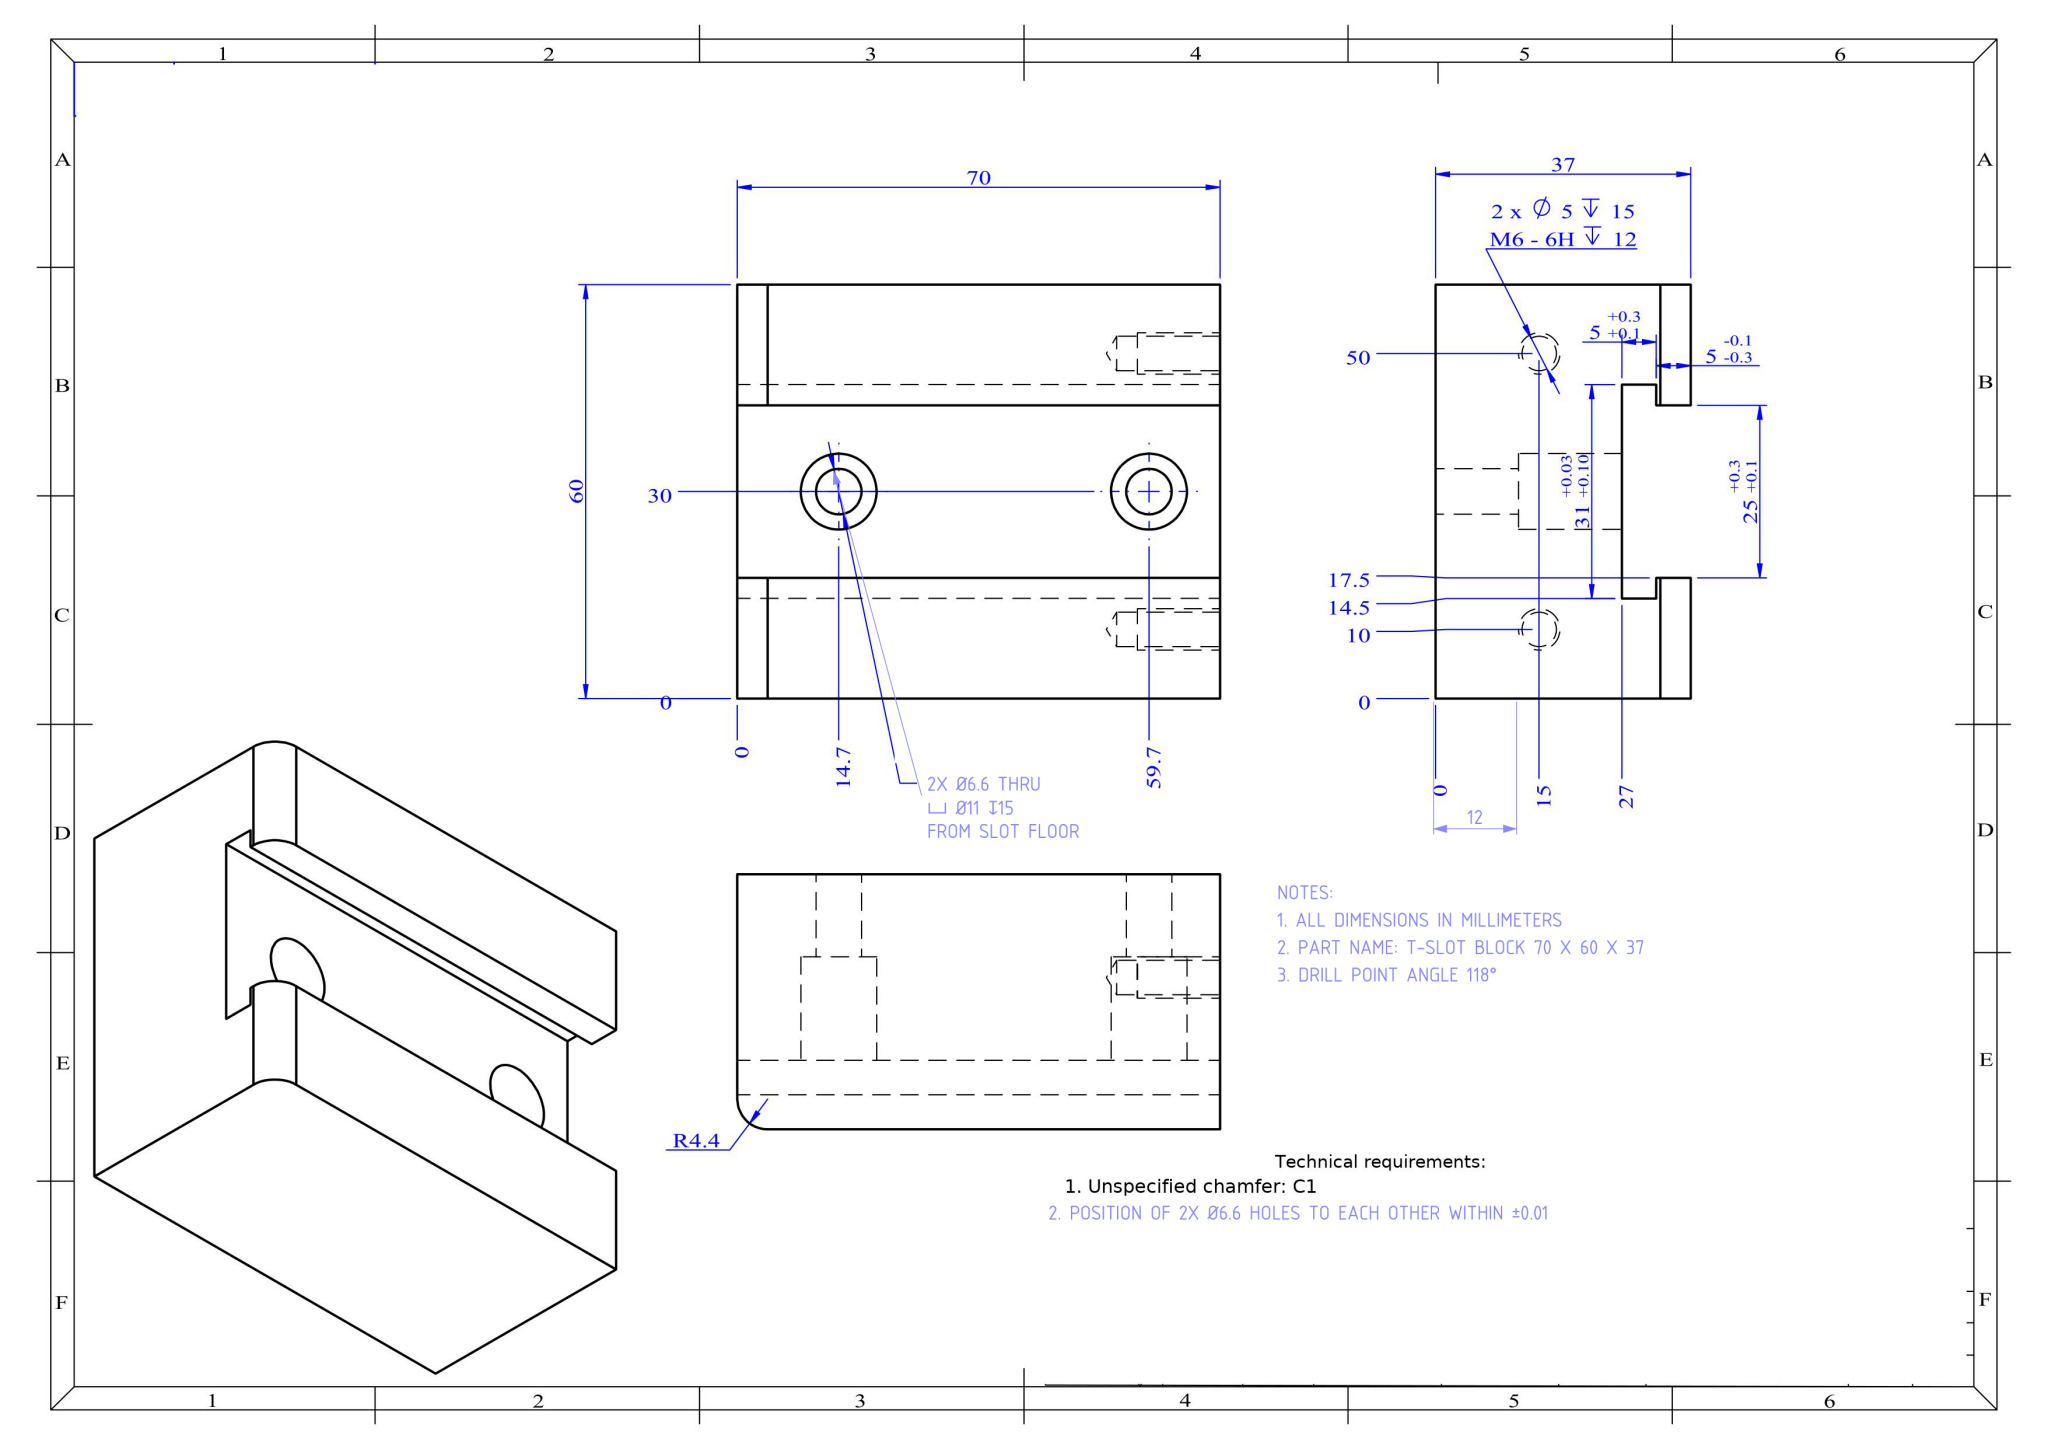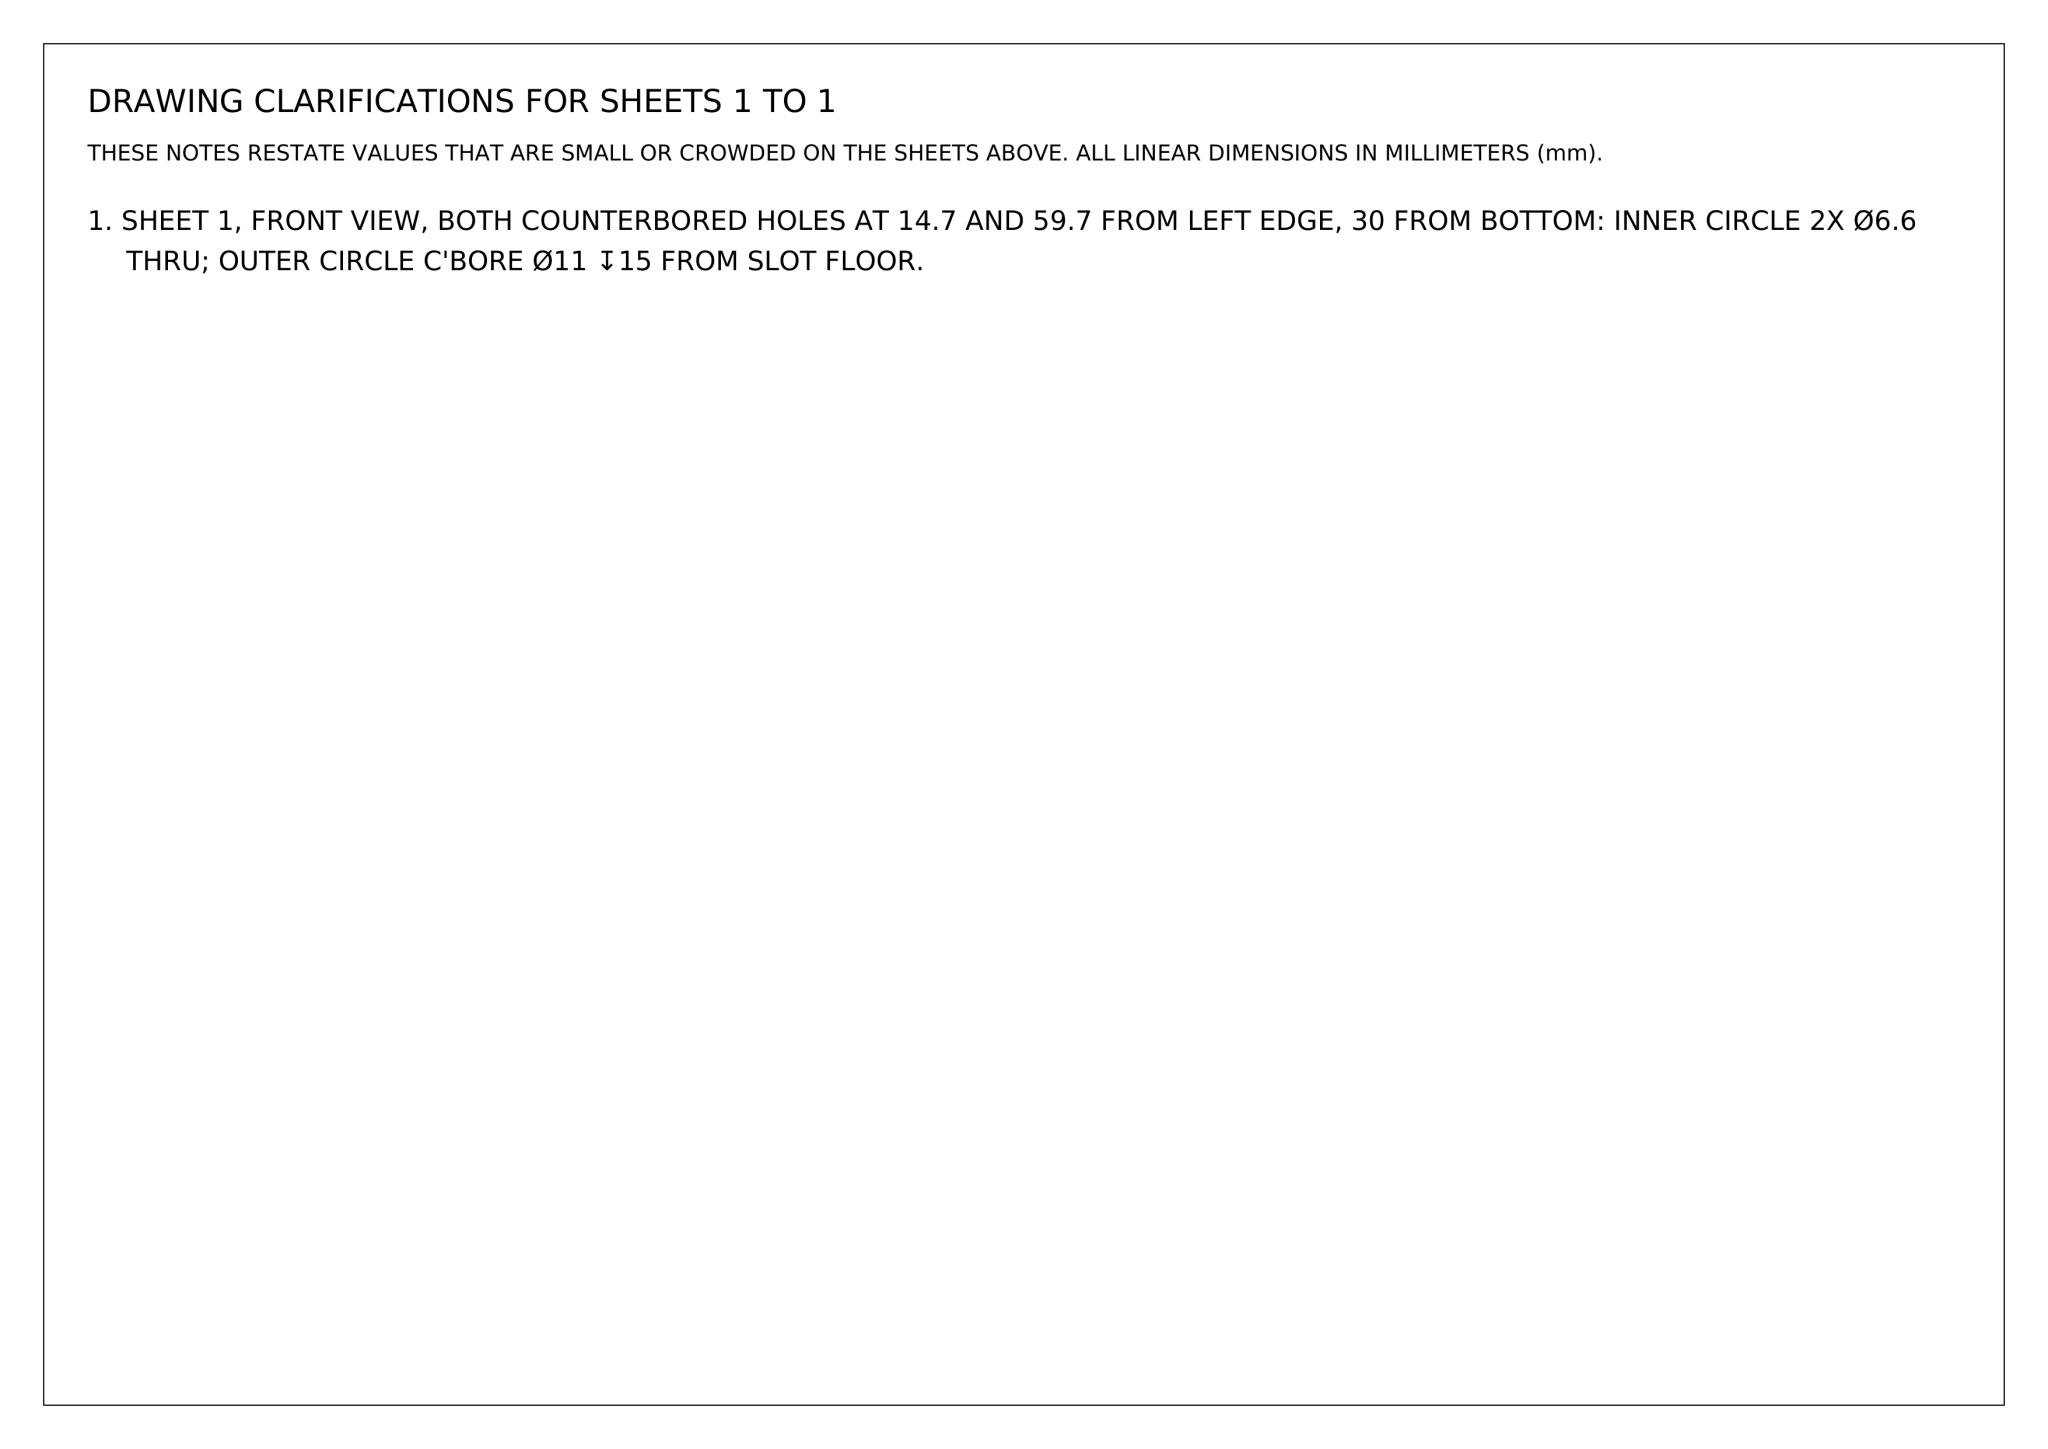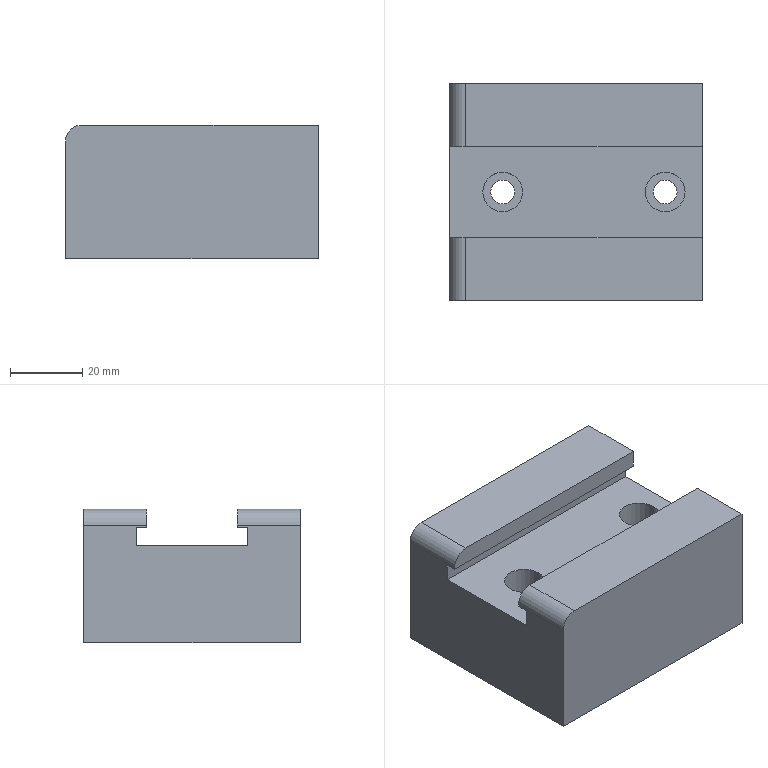Part | NX | mm | 1 solid | 34 faces | box 70 x 60 x 37 mm | volume 131374 mm3 | plane 16 | cylinder 14 | cone 4 | commonest cylinder face diameters 6.6 x4 11 x4 5 x4 8.8 x2